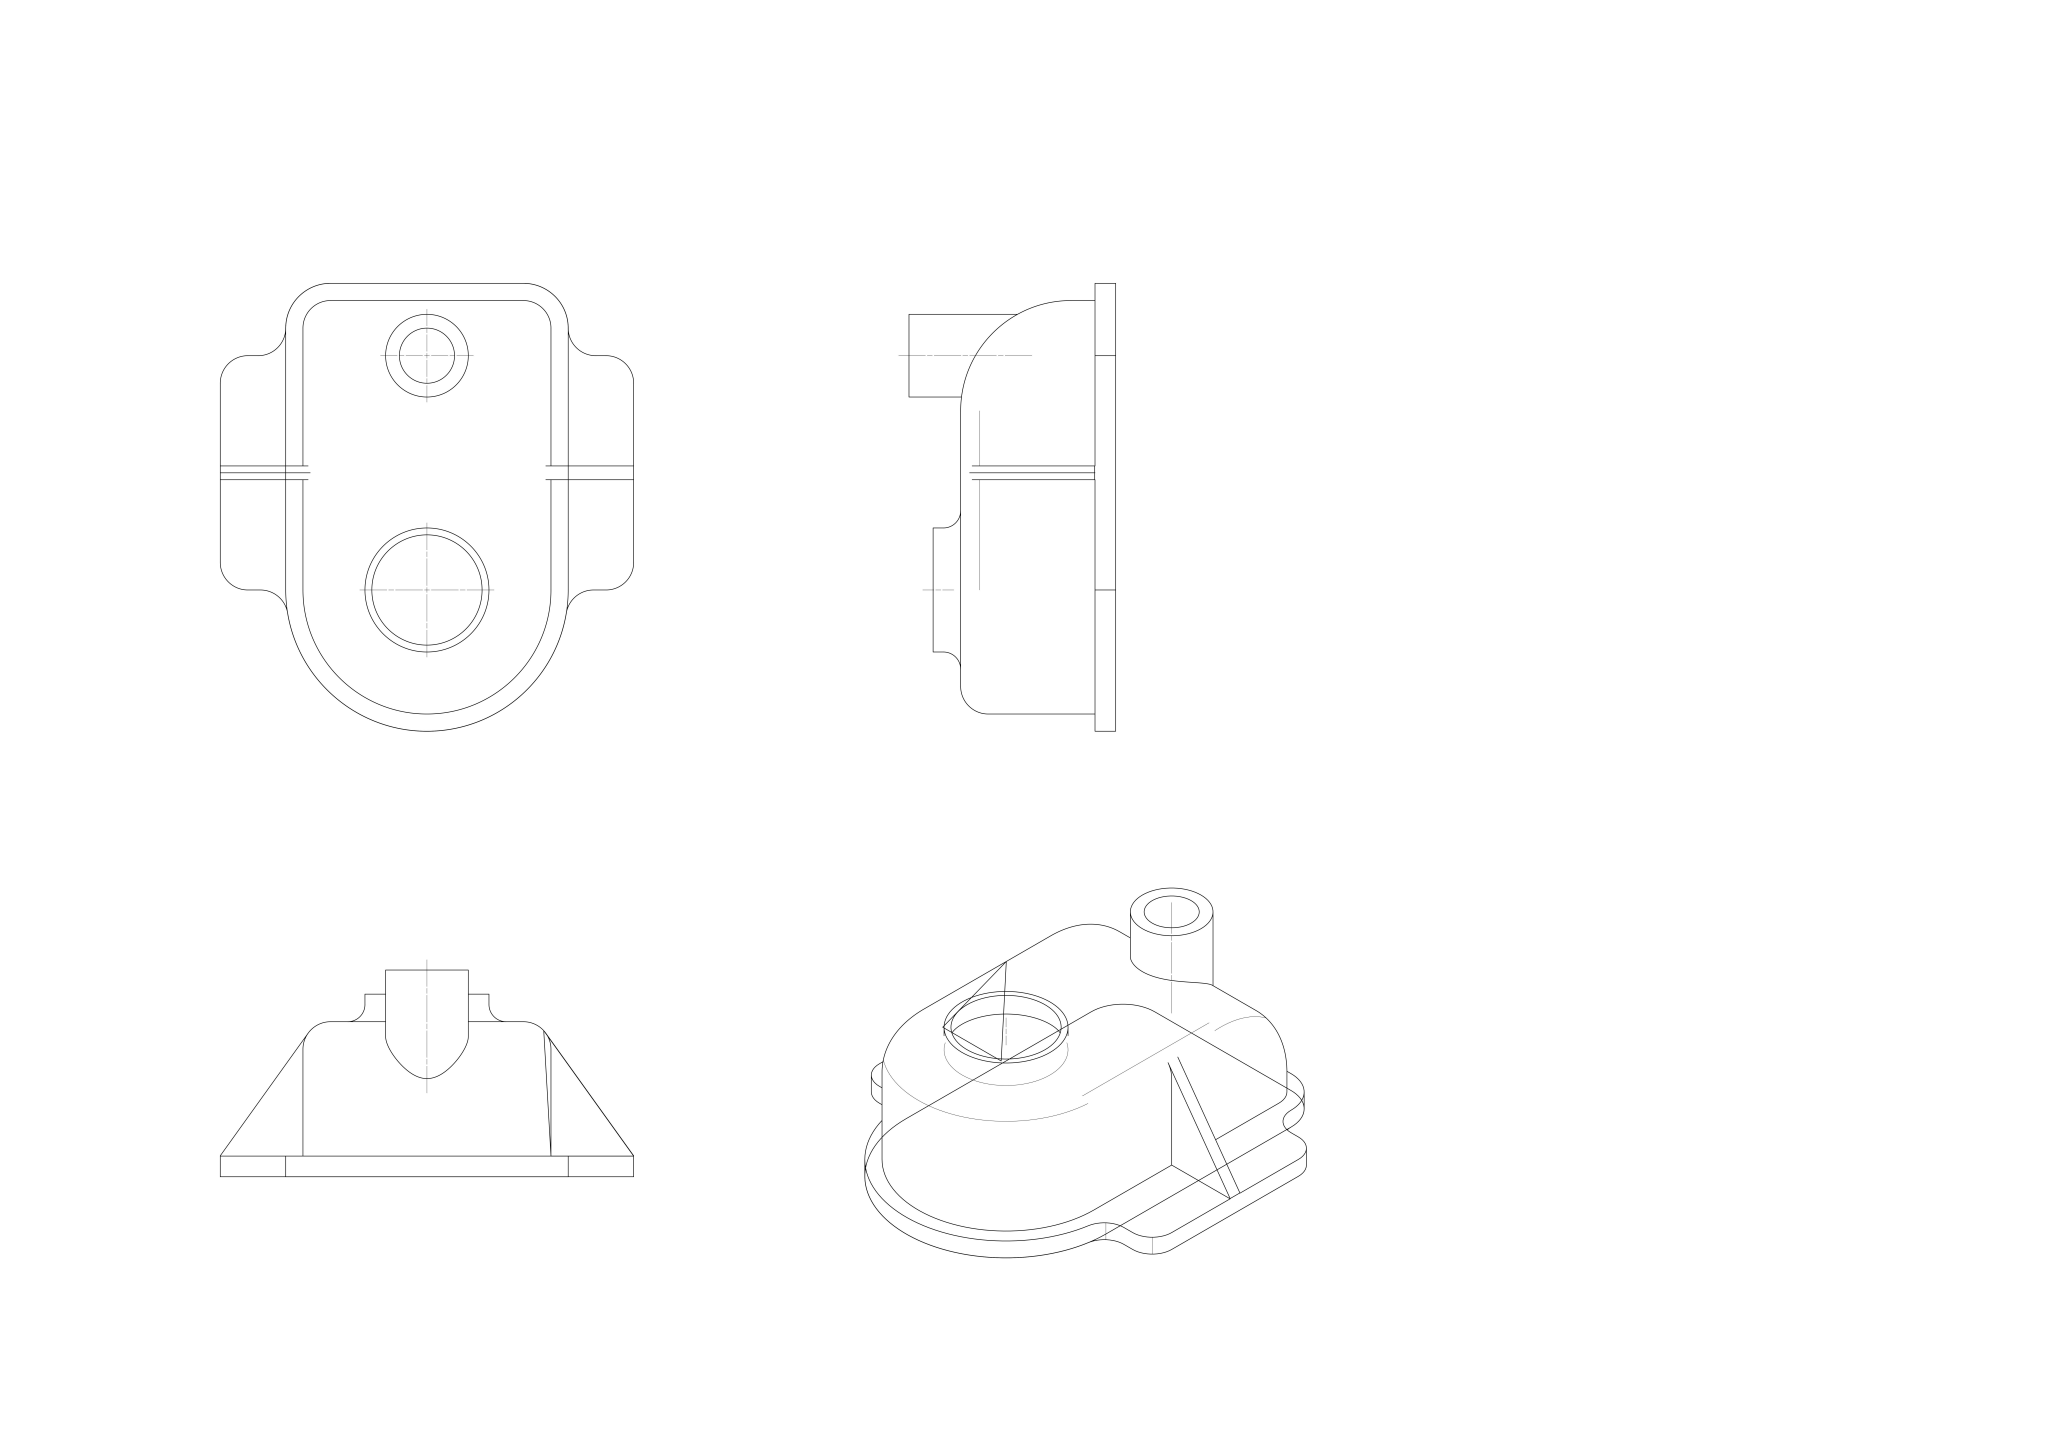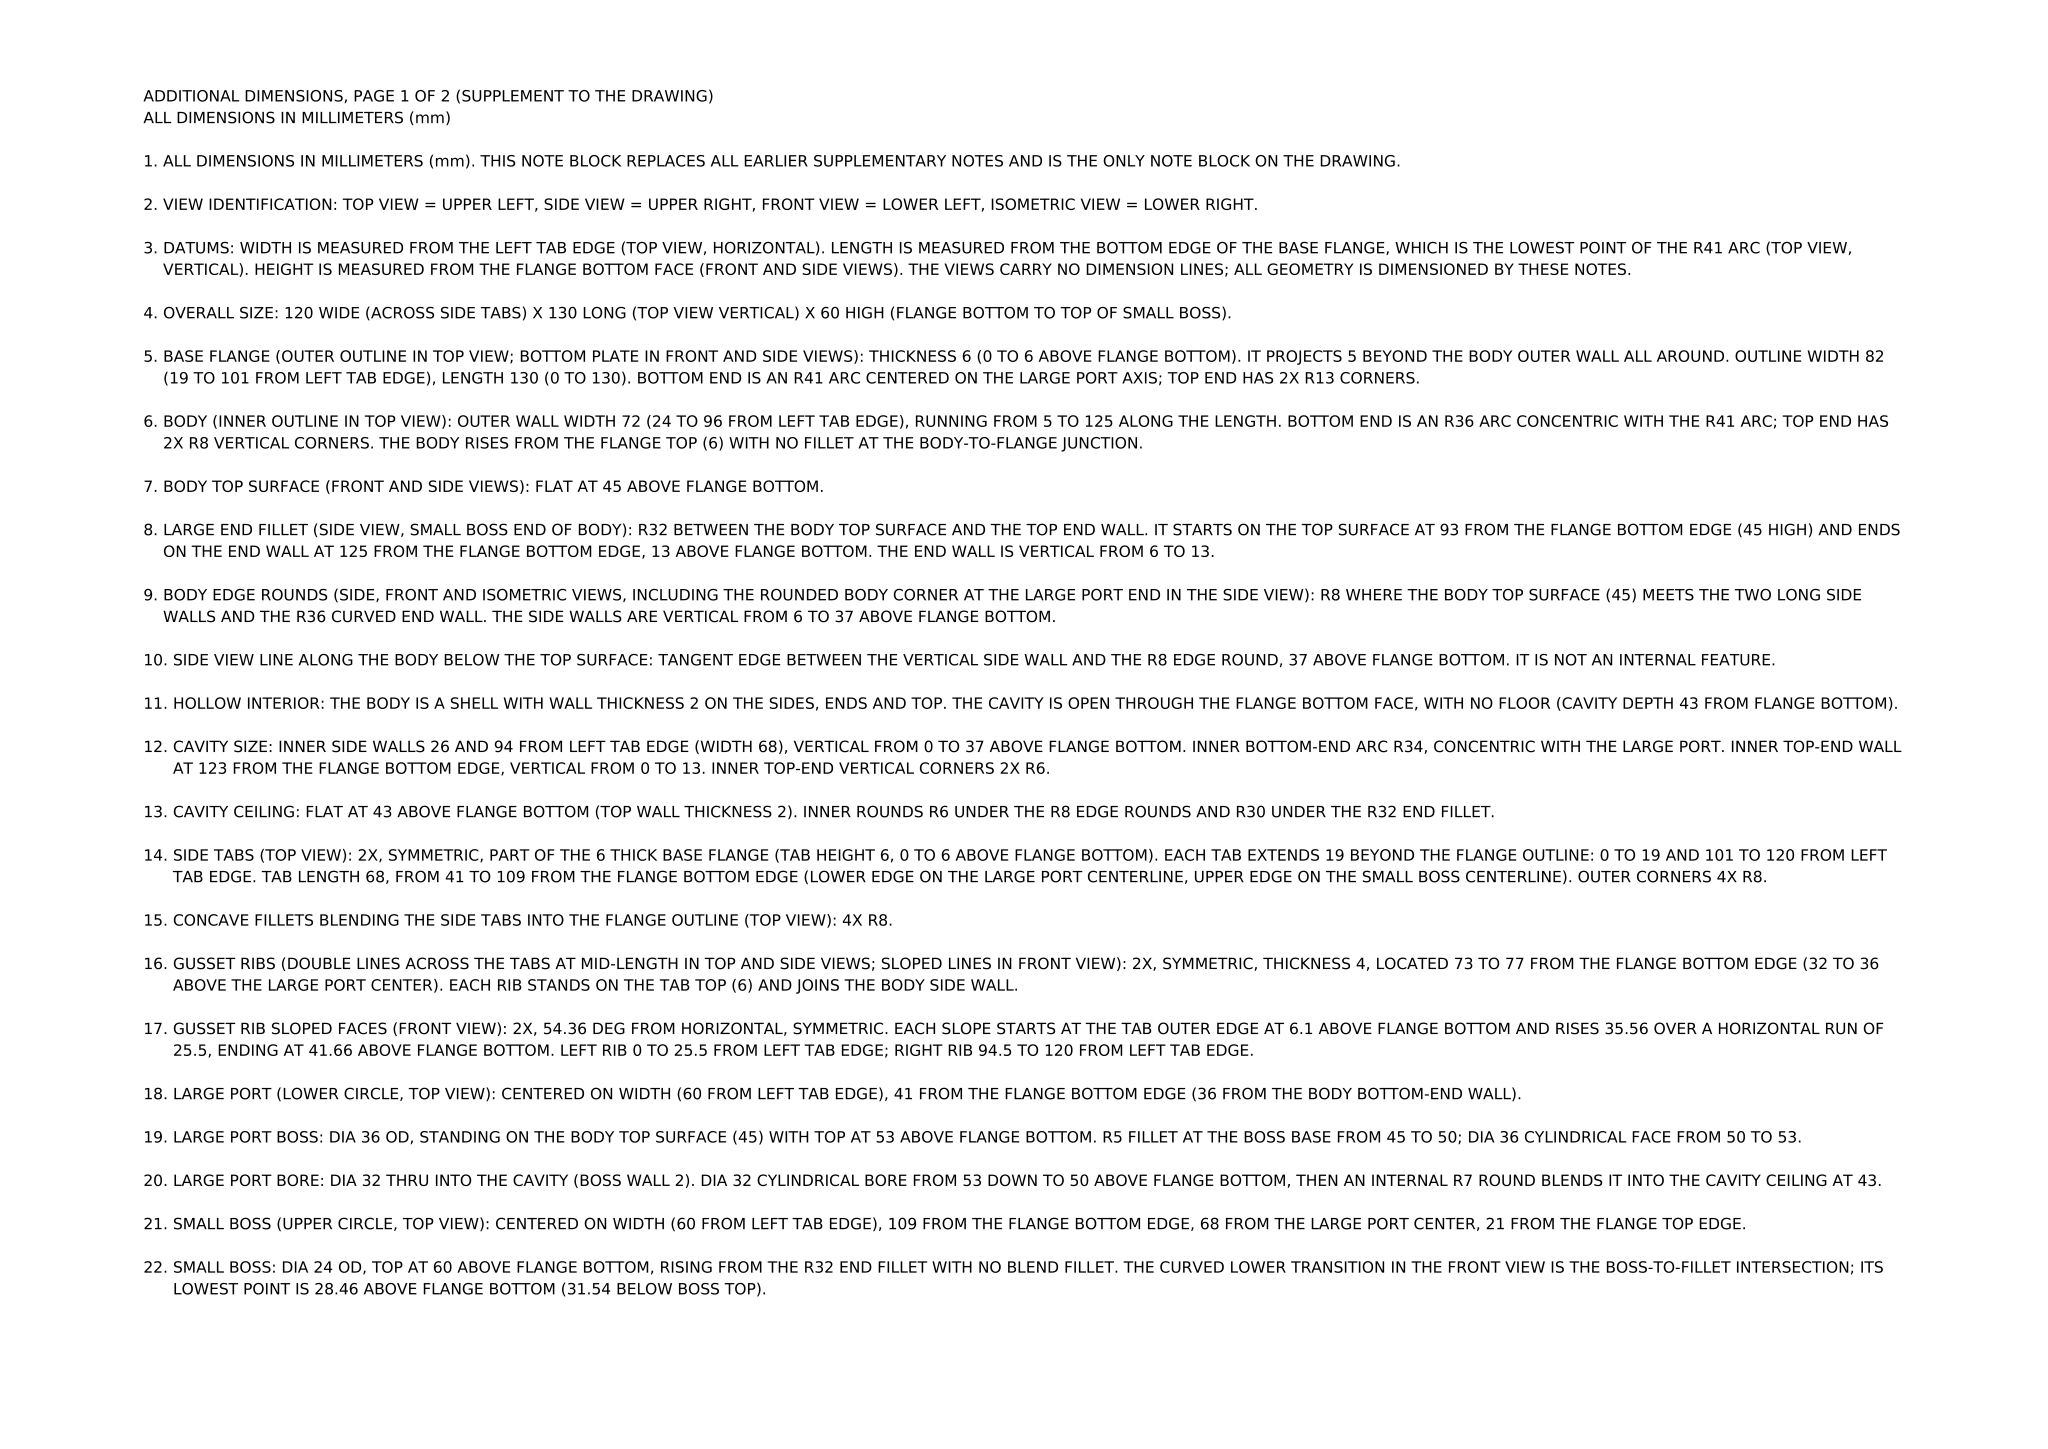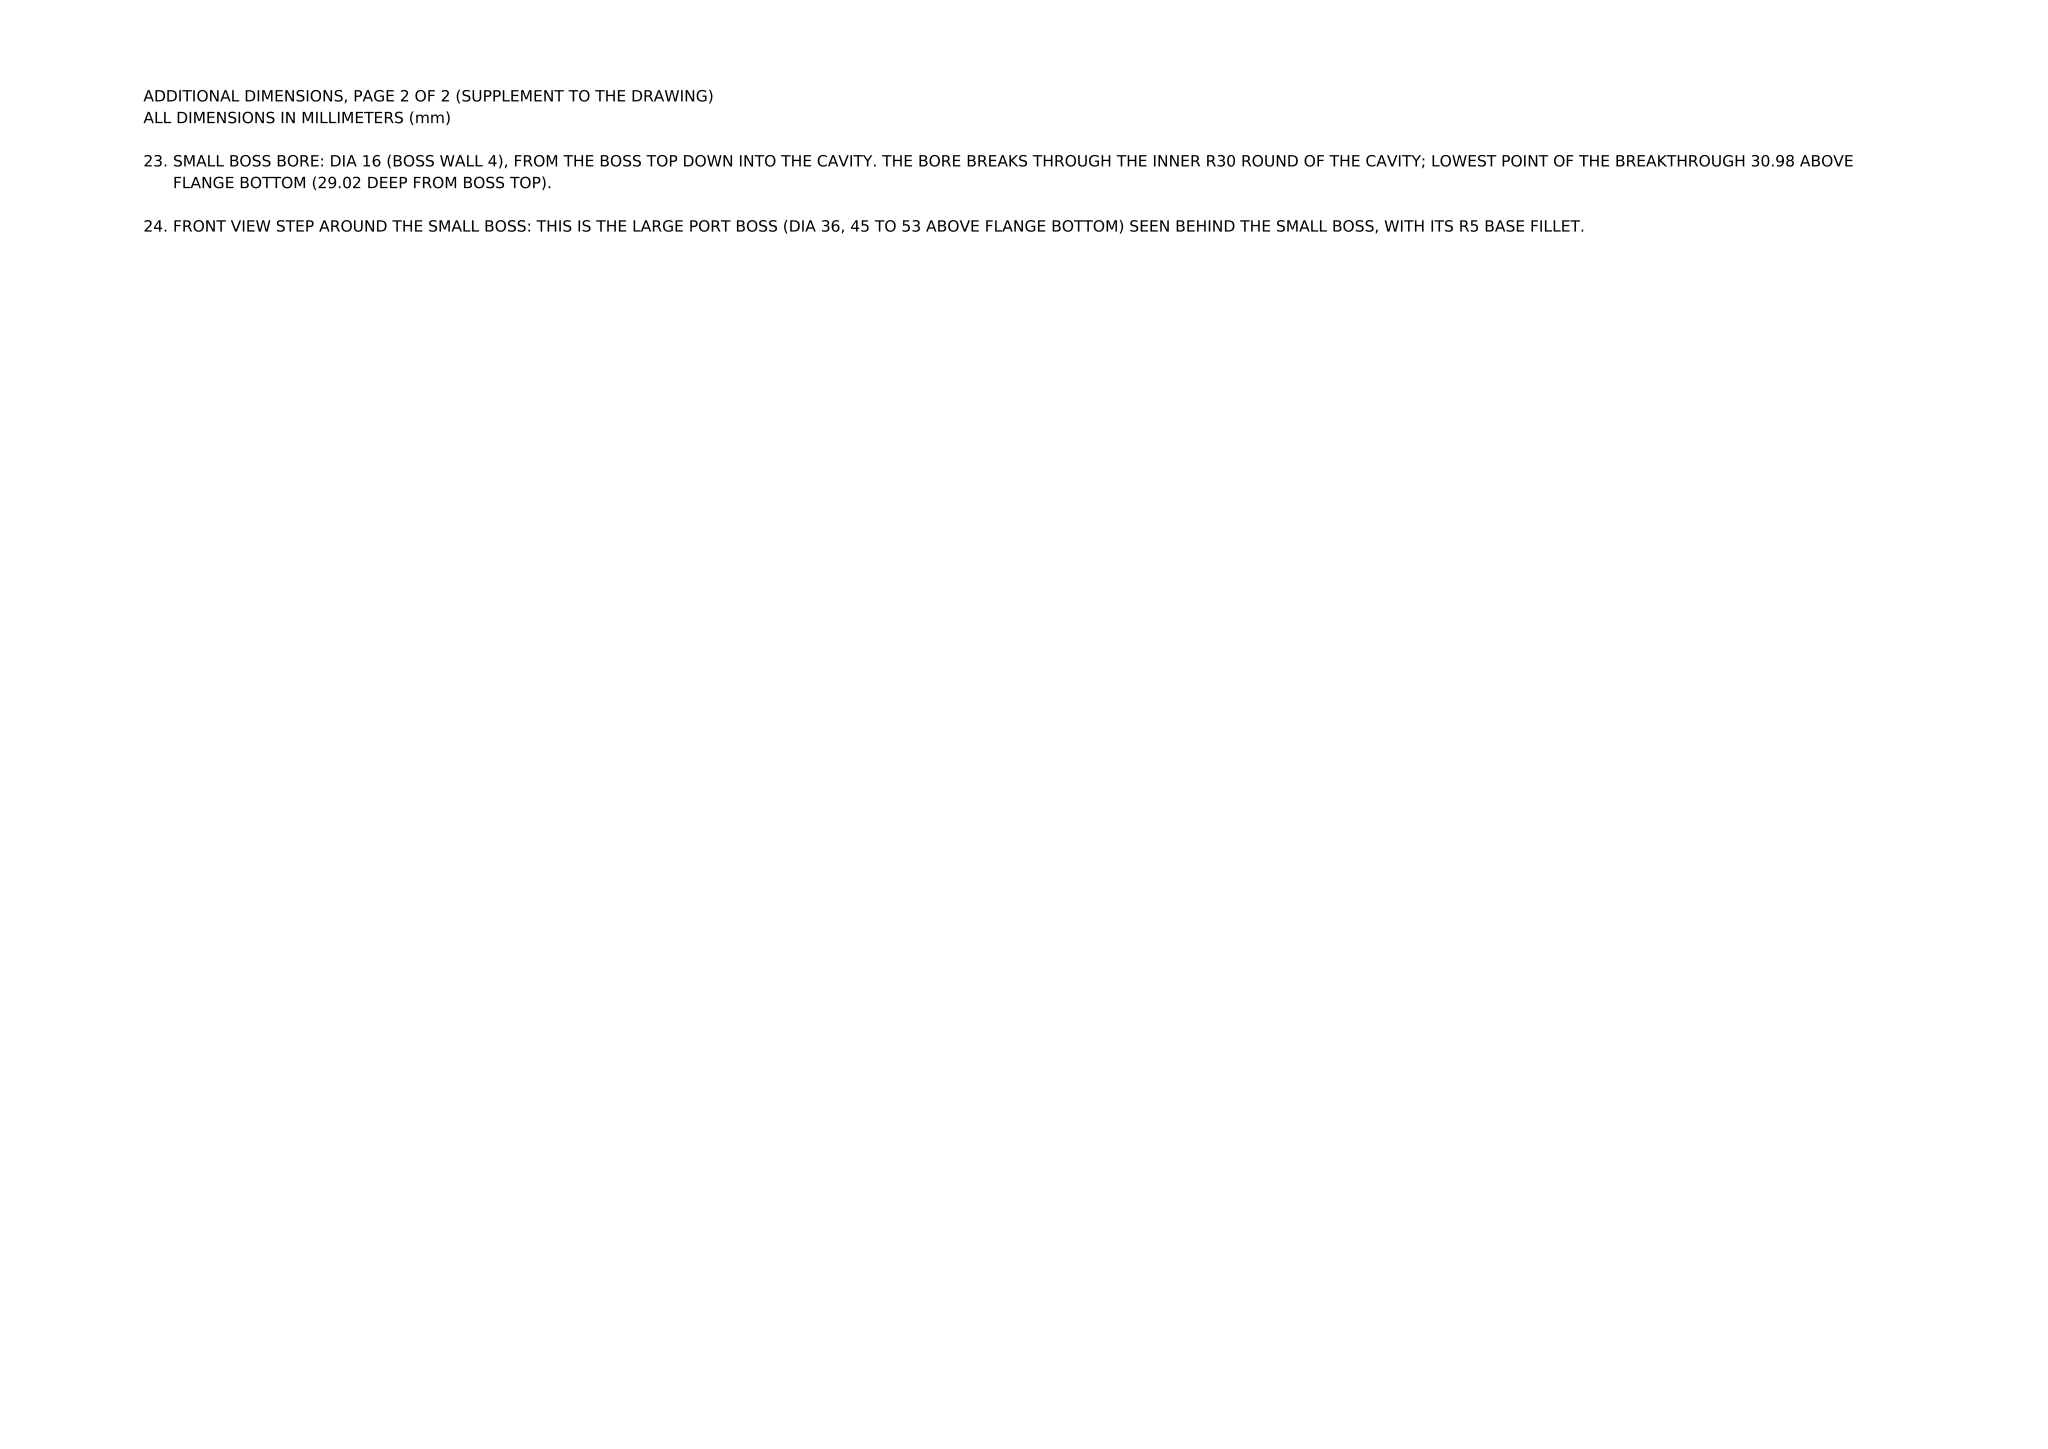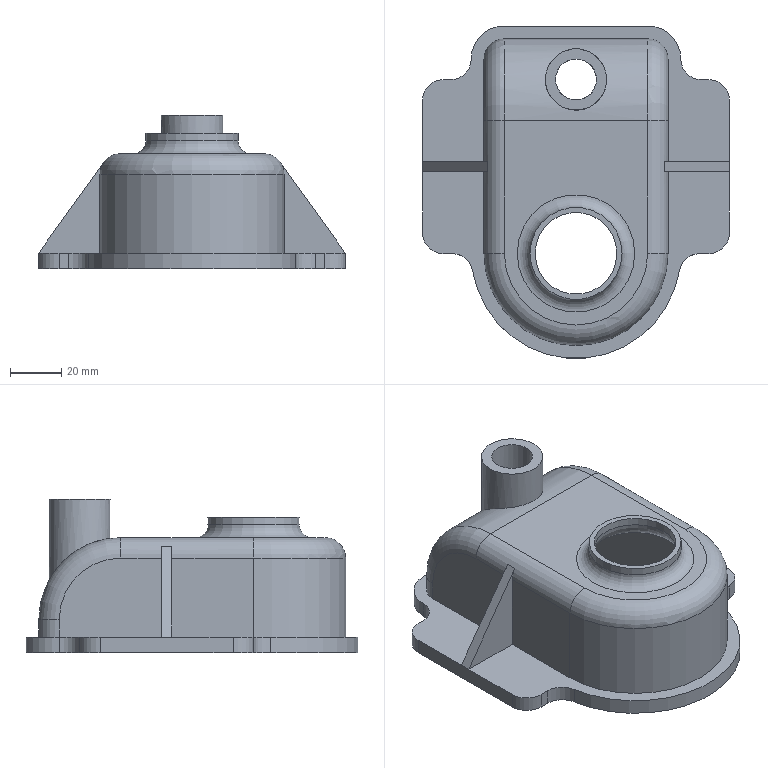Part | NX | mm | 1 solid | 63 faces | box 120 x 130 x 60 mm | volume 75010 mm3 | plane 28 | cylinder 27 | torus 8 | commonest cylinder face diameters 16 x13 12 x4 26 x2 72 x1 36 x1 64 x1 24 x1 32 x1